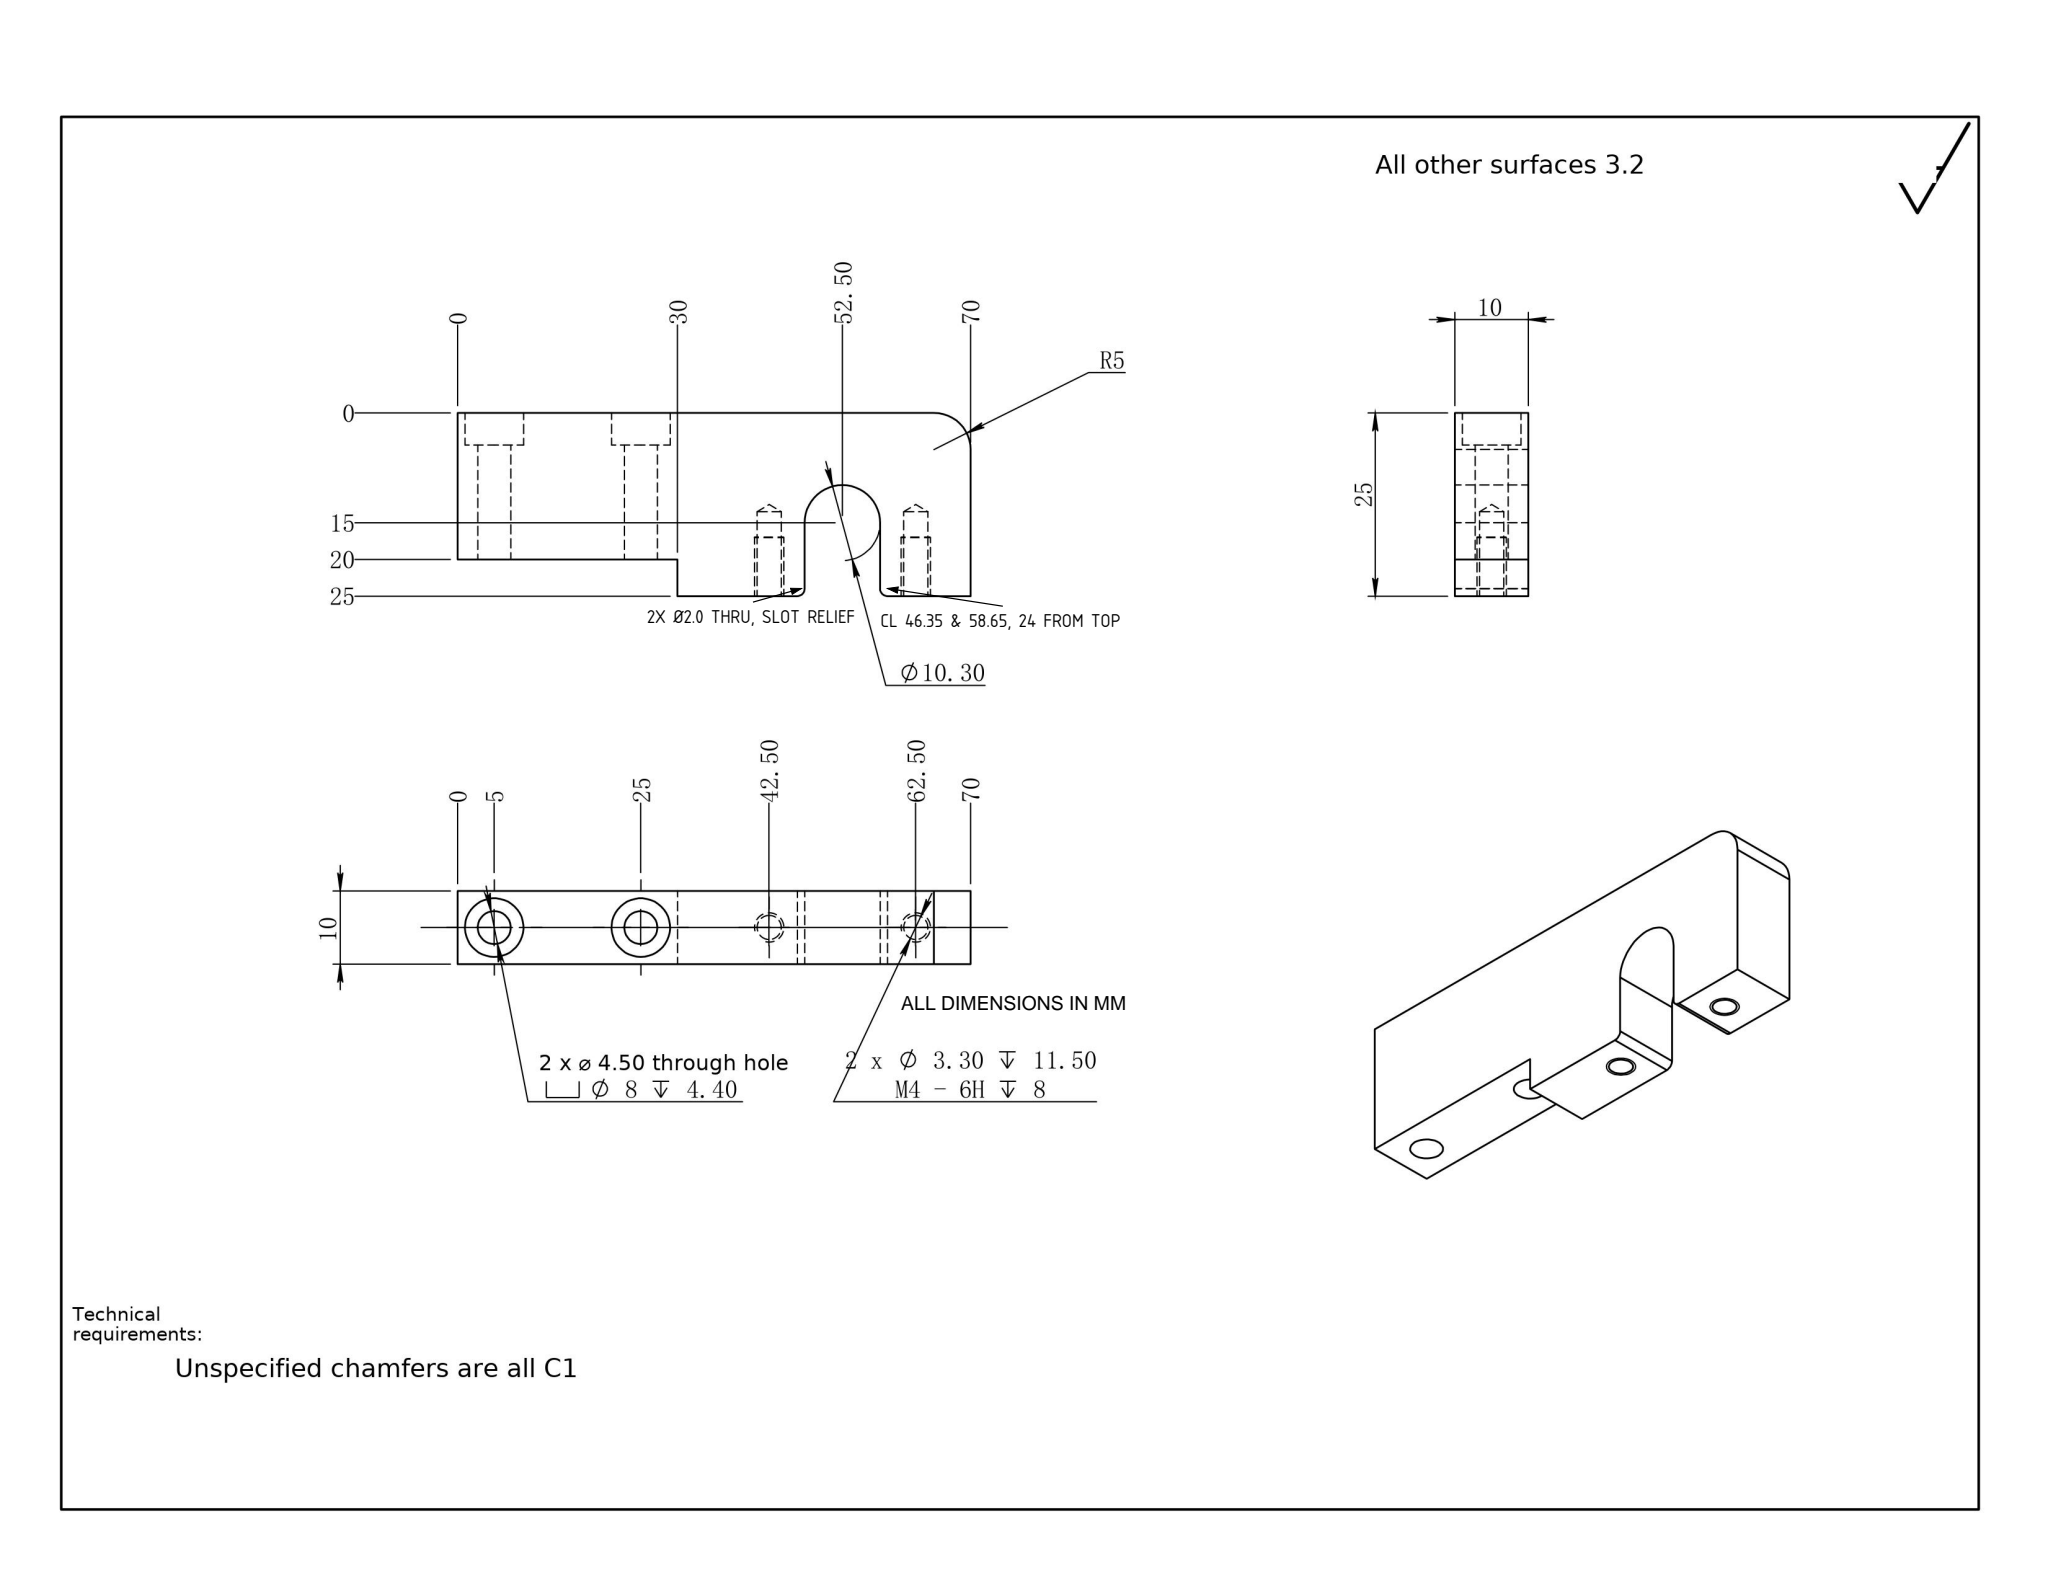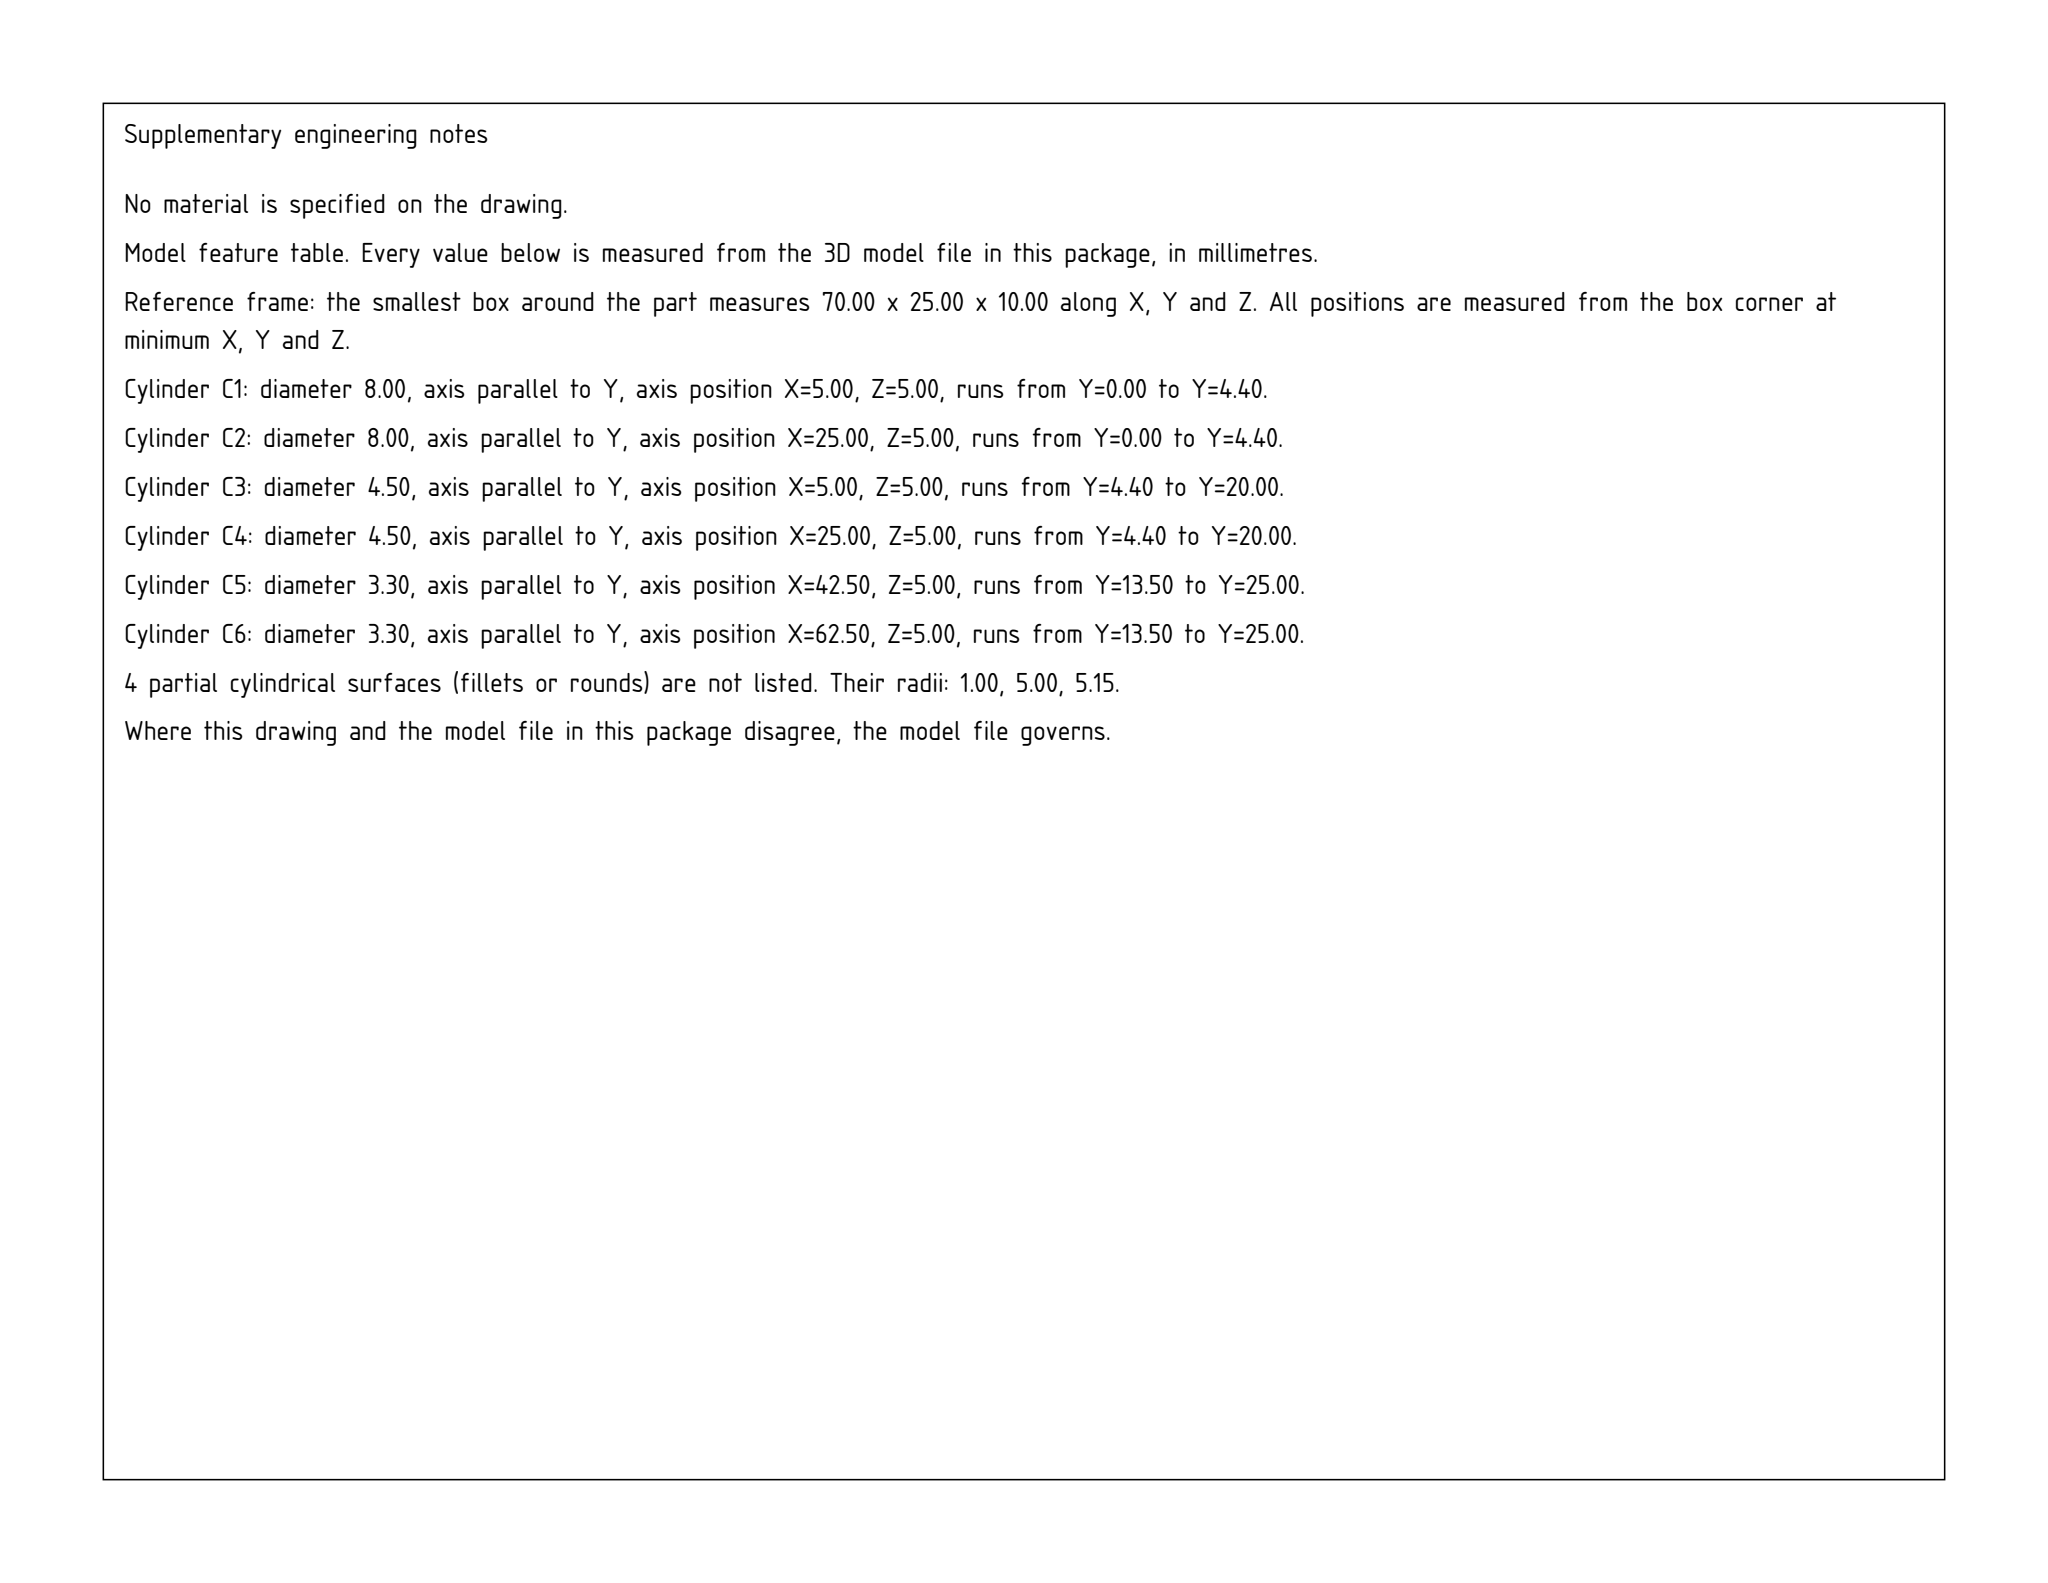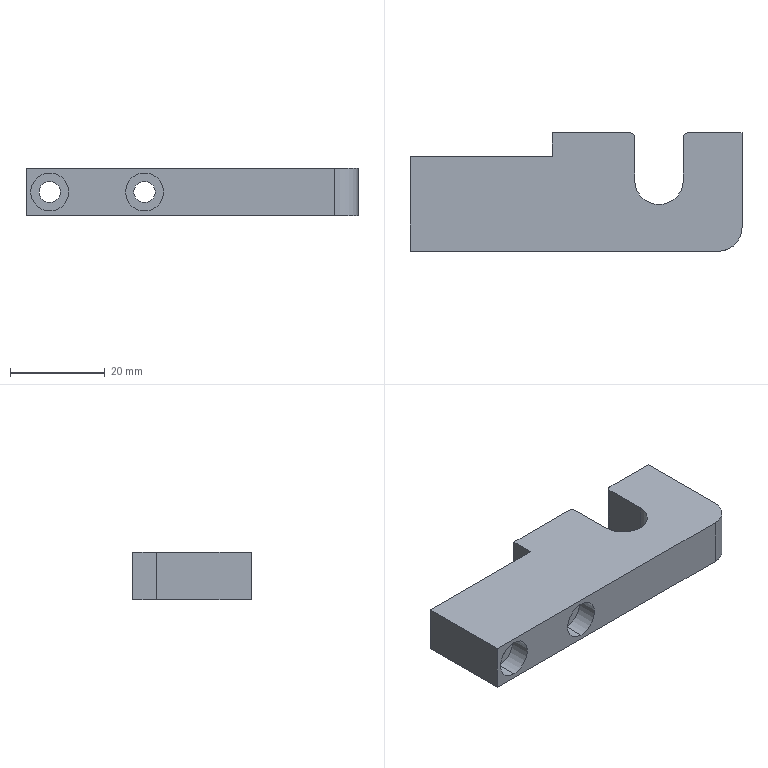Part | SolidWorks | mm | 1 solid | 33 faces | box 70 x 25 x 10 mm | volume 13355 mm3 | cylinder 16 | plane 13 | cone 4 | commonest cylinder face diameters 3.3 x4 8 x4 4.5 x4 2 x2 10.3 x1 10 x1
Drawing notes:
2 X Ø2.0 THRU (10 DEEP), SLOT CORNER RELIEF HOLES | from the solid: cylinders dia 2.0 axis z, length 10.0 = full 10 mm thickness, 2 off
Ø2.0 HOLE CL: X=46.35 & 58.65 FROM 0; 24 FROM TOP (0) FACE | from the solid: cyl dia 2.0 axis z at [46.35,24.0] and [58.65,24.0]; bbox y 0-25, slot walls x=47.35/57.65
build123d program:
from build123d import *

# Parameters (mm, degrees)
SKETCH1_W                                       = 70
SKETCH1_H                                       = 25
BOSS_EXTRUDE1_DEPTH                             = 5
SKETCH2_W                                       = 30
SKETCH2_H                                       = 5
CUT_EXTRUDE1_DEPTH                              = 39.487
SKETCH3_R                                       = 5.15
CUT_EXTRUDE2_DEPTH                              = 10
M4_HEX_SOCKET_HEAD_CAP_SCREW_CBORE1_D           = 4.5
M4_HEX_SOCKET_HEAD_CAP_SCREW_CBORE1_CBORE_D     = 8
M4_HEX_SOCKET_HEAD_CAP_SCREW_CBORE1_CBORE_DEPTH = 4.4
CUT_EXTRUDE3_DEPTH                              = 39.487
M4_TAPPED_HOLE1_D                               = 3.3
M4_TAPPED_HOLE1_DEPTH                           = 11.5
M4_TAPPED_HOLE1_TIP                             = 0.9914
FILLET1_R                                       = 1
FILLET2_R                                       = 5


with BuildPart() as part:
    # Sketch1 → Boss-Extrude1 (new, symmetric)
    with BuildSketch(Plane.XY):
        Rectangle(SKETCH1_W, SKETCH1_H)
    extrude(amount=BOSS_EXTRUDE1_DEPTH, both=True)

    # Sketch2 → Cut-Extrude1 (cut, through all)
    with BuildSketch(Plane.XY.offset(5)):
        with Locations((-20, 10)):
            Rectangle(SKETCH2_W, SKETCH2_H)
    extrude(amount=-CUT_EXTRUDE1_DEPTH, mode=Mode.SUBTRACT)

    # Sketch3 → Cut-Extrude2 (cut)
    with BuildSketch(Plane.XY.offset(5)):
        with Locations((17.5, 2.5)):
            Circle(SKETCH3_R)
    extrude(amount=-CUT_EXTRUDE2_DEPTH, mode=Mode.SUBTRACT)

    # M4 Hex Socket Head Cap Screw CBORE1 (through all)
    with Locations(Plane(origin=(0, -12.5, 0), x_dir=(-1, 0, 0), z_dir=(0, -1, 0))):
        with Locations((30, 0), (10, 0)):
            CounterBoreHole(M4_HEX_SOCKET_HEAD_CAP_SCREW_CBORE1_D / 2, M4_HEX_SOCKET_HEAD_CAP_SCREW_CBORE1_CBORE_D / 2, M4_HEX_SOCKET_HEAD_CAP_SCREW_CBORE1_CBORE_DEPTH)

    # Sketch6 → Cut-Extrude3 (cut, through all)
    with BuildSketch(Plane.XY.offset(5)):
        with BuildLine():
            Line((12.35, 2.5), (12.35, 12.5))
            ThreePointArc((12.35, 12.5), (17.5, 17.65), (22.65, 12.5))
            Line((22.65, 12.5), (22.65, 2.5))
            ThreePointArc((22.65, 2.5), (17.5, -2.65), (12.35, 2.5))
        make_face()
    extrude(amount=-CUT_EXTRUDE3_DEPTH, mode=Mode.SUBTRACT)

    # M4 Tapped Hole1
    with Locations(Plane(origin=(0, 12.5, 0), x_dir=(1, 0, 0), z_dir=(0, 1, 0))):
        with Locations((7.5, 0), (27.5, 0)):
            Hole(M4_TAPPED_HOLE1_D / 2, depth=M4_TAPPED_HOLE1_DEPTH)
            with Locations((0, 0, -(M4_TAPPED_HOLE1_DEPTH + M4_TAPPED_HOLE1_TIP / 2))):  # 118° drill point
                Cone(0, M4_TAPPED_HOLE1_D / 2, M4_TAPPED_HOLE1_TIP, mode=Mode.SUBTRACT)

    # Fillet1
    fillet1_edges = [part.edges().sort_by_distance(p)[0] for p in [
        (12.35, 12.5, 0),
        (22.65, 12.5, 0),
    ]]
    fillet(fillet1_edges, radius=FILLET1_R)

    # Fillet2
    fillet2_edges = [part.edges().sort_by_distance(p)[0] for p in [
        (35, -12.5, 0),
    ]]
    fillet(fillet2_edges, radius=FILLET2_R)


solid = part.part